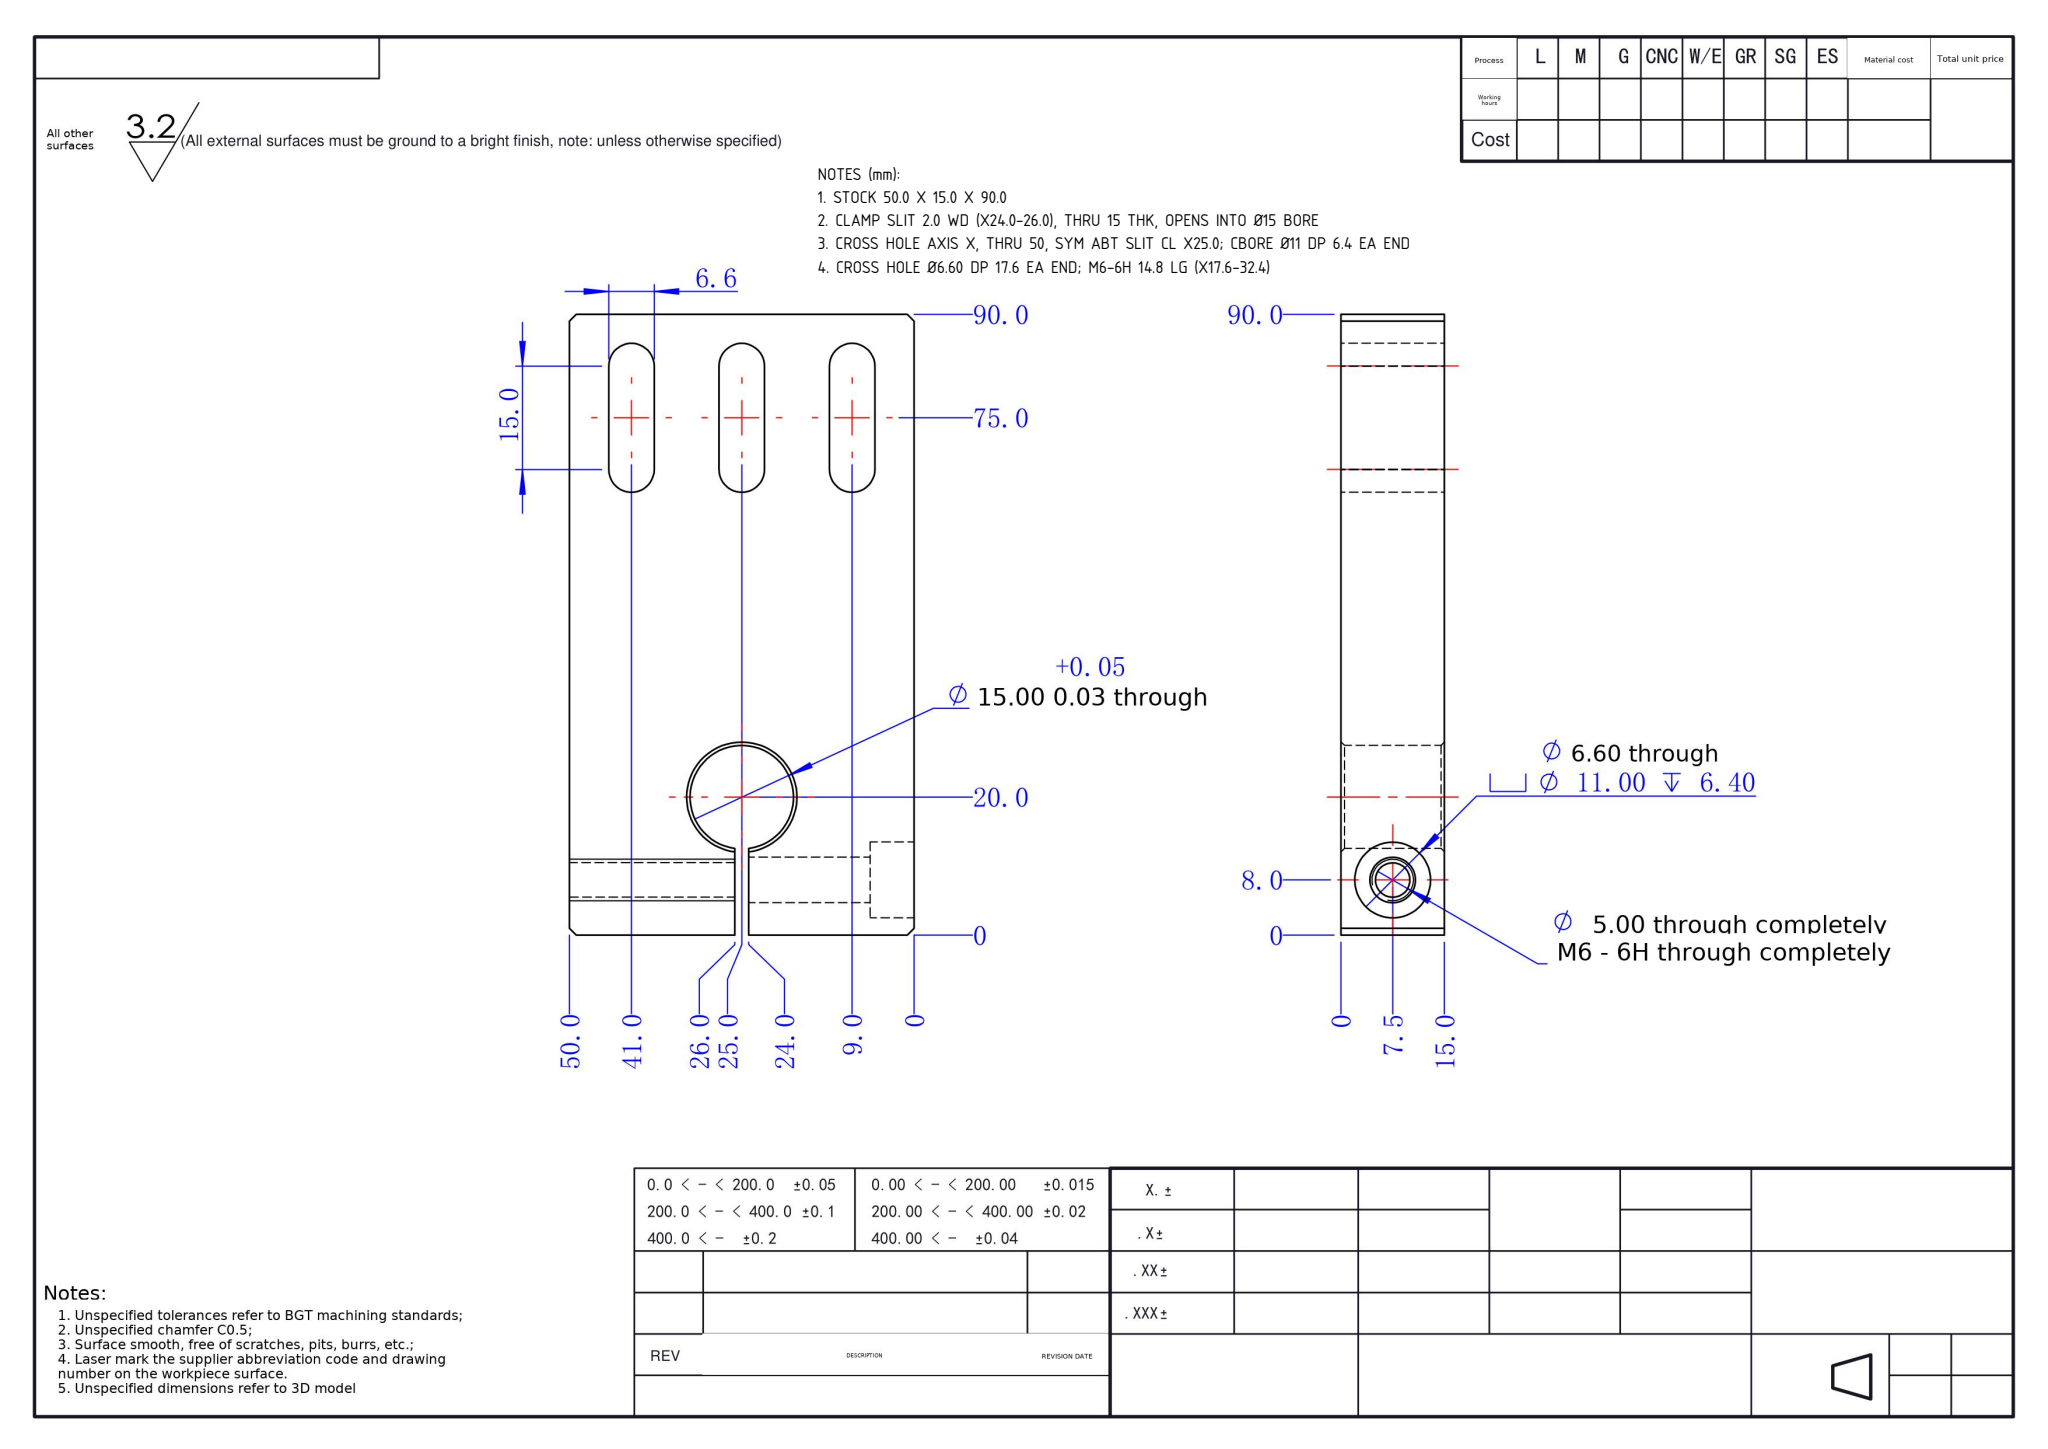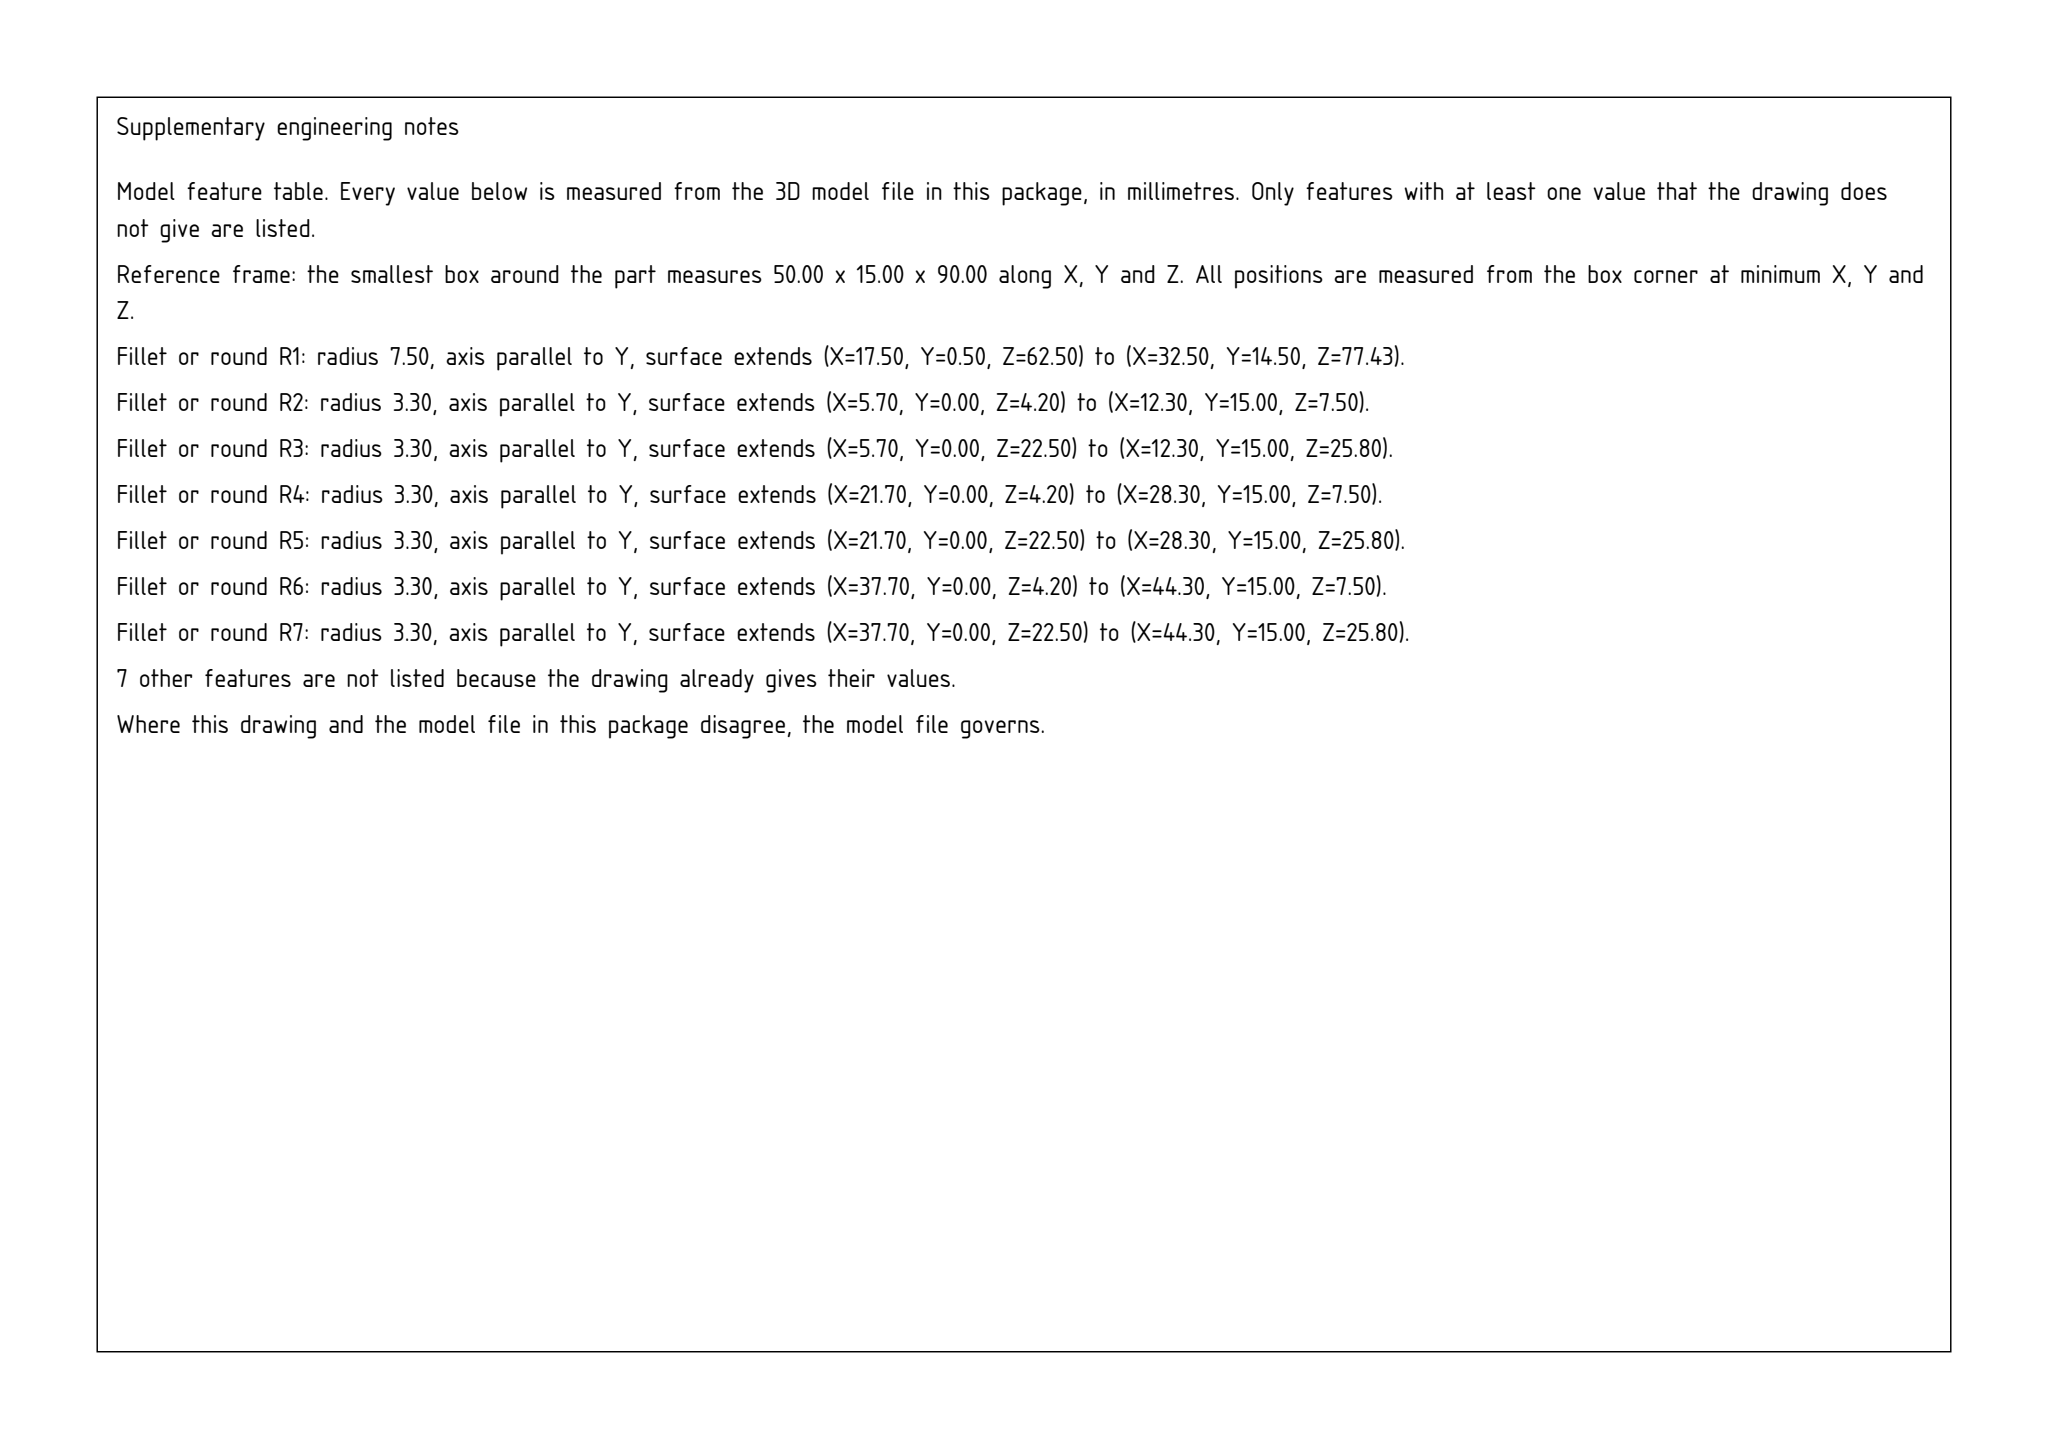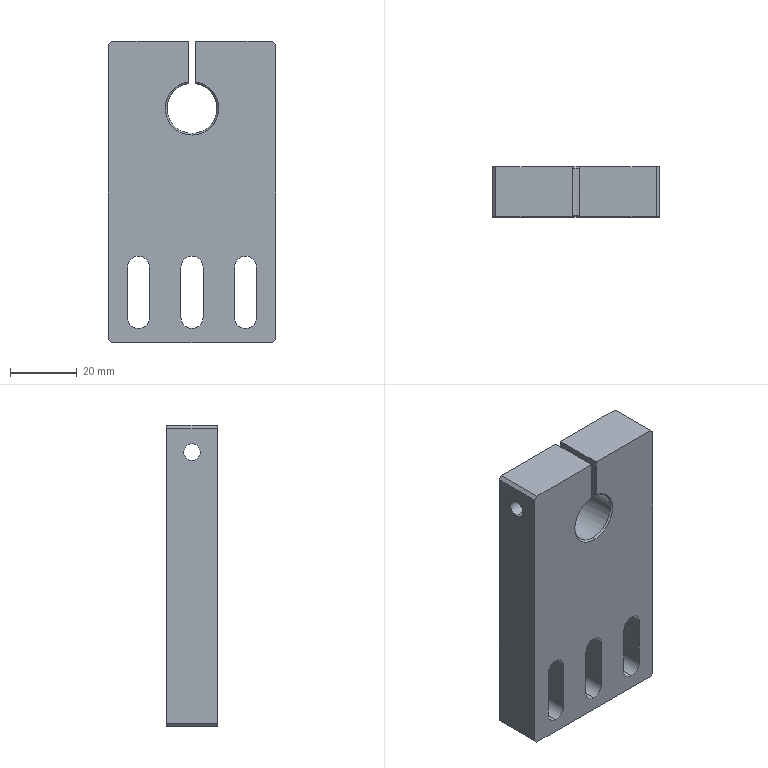Part | SolidWorks | mm | 1 solid | 39 faces | box 50 x 15 x 90 mm | volume 56756 mm3 | plane 20 | cylinder 16 | cone 3 | commonest cylinder face diameters 6.6 x11 5 x2 11 x2 15 x1
Drawing notes:
STOCK 50.0 X 15.0 X 90.0 | from the solid: bbox_xyz [50.0, 15.0, 90.0]
CLAMP SLIT 2.0 WD (X24.0-26.0), THRU 15 THK, OPENS INTO Ø15 BORE | from the solid: axis_planes x=24.0 & x=26.0 (2.0 gap); y planes 0 & 15 thru; Ø15 bore axis y, pos x=25.0
CROSS HOLE AXIS X, THRU 50, SYM ABT SLIT CL X25.0; CBORE Ø11 DP 6.4 EA END | from the solid: cylinders Ø5.0/Ø6.6/Ø11.0 axis x at y=7.5, count 2 ea end; Ø11 L=6.4; bbox x=50; slit CL x=25.0
CROSS HOLE Ø6.60 DP 17.6 EA END; M6-6H 14.8 LG (X17.6-32.4) | from the solid: Ø6.6 x-axis cyls L=17.6 at x0-17.6 and x32.4-50; Ø5 tap drill spans middle 14.8
build123d program:
from build123d import *

# Parameters (mm, degrees)
SKETCH1_W                                       = 50
SKETCH1_H                                       = 90
BOSS_EXTRUDE1_DEPTH                             = 15
SKETCH2_R                                       = 7.5
CUT_EXTRUDE1_DEPTH                              = 105.043
SKETCH3_W                                       = 2
SKETCH3_H                                       = 18.433
CUT_EXTRUDE2_DEPTH                              = 105.043
M6_HEX_SOCKET_HEAD_CAP_SCREW_CBORE1_D           = 6.6
M6_HEX_SOCKET_HEAD_CAP_SCREW_CBORE1_DEPTH       = 24
M6_HEX_SOCKET_HEAD_CAP_SCREW_CBORE1_CBORE_D     = 11
M6_HEX_SOCKET_HEAD_CAP_SCREW_CBORE1_CBORE_DEPTH = 6.4
M6_TAPPED_HOLE1_D                               = 5
CUT_EXTRUDE3_DEPTH                              = 105.043
CHAMFER1_SIZE                                   = 1
CHAMFER2_SIZE                                   = 0.5


with BuildPart() as part:
    # Sketch1 → Boss-Extrude1 (new body)
    with BuildSketch(Plane(origin=(0, 0, 0), x_dir=(1, 0, 0), z_dir=(0, 1, 0))):
        with Locations((25, 45)):
            Rectangle(SKETCH1_W, SKETCH1_H)
    extrude(amount=BOSS_EXTRUDE1_DEPTH)

    # Sketch2 → Cut-Extrude1 (cut, through all)
    with BuildSketch(Plane(origin=(0, 15, 0), x_dir=(1, 0, 0), z_dir=(0, 1, 0))):
        with Locations(Location((25, 20, 0), (0, 0, 270))):
            Circle(SKETCH2_R)
    extrude(amount=-CUT_EXTRUDE1_DEPTH, mode=Mode.SUBTRACT)

    # Sketch3 → Cut-Extrude2 (cut, through all)
    with BuildSketch(Plane(origin=(0, 15, 0), x_dir=(1, 0, 0), z_dir=(0, 1, 0))):
        with Locations((25, 9.216)):
            Rectangle(SKETCH3_W, SKETCH3_H)
    extrude(amount=-CUT_EXTRUDE2_DEPTH, mode=Mode.SUBTRACT)

    # M6 Hex Socket Head Cap Screw CBORE1
    with Locations(Plane(origin=(50, 0, 0), x_dir=(0, 0, -1), z_dir=(1, 0, 0))):
        with Locations((8, 7.5)):
            CounterBoreHole(M6_HEX_SOCKET_HEAD_CAP_SCREW_CBORE1_D / 2, M6_HEX_SOCKET_HEAD_CAP_SCREW_CBORE1_CBORE_D / 2, M6_HEX_SOCKET_HEAD_CAP_SCREW_CBORE1_CBORE_DEPTH, depth=M6_HEX_SOCKET_HEAD_CAP_SCREW_CBORE1_DEPTH)

    # M6 Tapped Hole1 (through all)
    with Locations(Plane(origin=(24, 0, 0), x_dir=(0, 0, -1), z_dir=(1, 0, 0))):
        with Locations((8, 7.5)):
            Hole(M6_TAPPED_HOLE1_D / 2)

    # Sketch9 → Cut-Extrude3 (cut, through all)
    with BuildSketch(Plane.XZ):
        with BuildLine():
            Line((12.3, -67.5), (12.3, -82.5))
            ThreePointArc((12.3, -82.5), (9, -85.8), (5.7, -82.5))
            Line((5.7, -82.5), (5.7, -67.5))
            ThreePointArc((5.7, -67.5), (9, -64.2), (12.3, -67.5))
        make_face()
        with BuildLine():
            Line((28.3, -67.5), (28.3, -82.5))
            ThreePointArc((28.3, -82.5), (25, -85.8), (21.7, -82.5))
            Line((21.7, -82.5), (21.7, -67.5))
            ThreePointArc((21.7, -67.5), (25, -64.2), (28.3, -67.5))
        make_face()
        with BuildLine():
            Line((44.3, -67.5), (44.3, -82.5))
            ThreePointArc((44.3, -82.5), (41, -85.8), (37.7, -82.5))
            Line((37.7, -82.5), (37.7, -67.5))
            ThreePointArc((37.7, -67.5), (41, -64.2), (44.3, -67.5))
        make_face()
    extrude(amount=-CUT_EXTRUDE3_DEPTH, mode=Mode.SUBTRACT)

    # Chamfer1
    chamfer1_edges = [part.edges().sort_by_distance(p)[0] for p in [
        (0, 7.5, -90),
        (50, 7.5, -90),
        (50, 7.5, 0),
        (0, 7.5, 0),
    ]]
    chamfer(chamfer1_edges, length=CHAMFER1_SIZE)

    # Chamfer2
    chamfer2_edges = [part.edges().sort_by_distance(p)[0] for p in [
        (25, 0, -27.5),
        (25, 15, -27.5),
    ]]
    chamfer(chamfer2_edges, length=CHAMFER2_SIZE)


solid = part.part